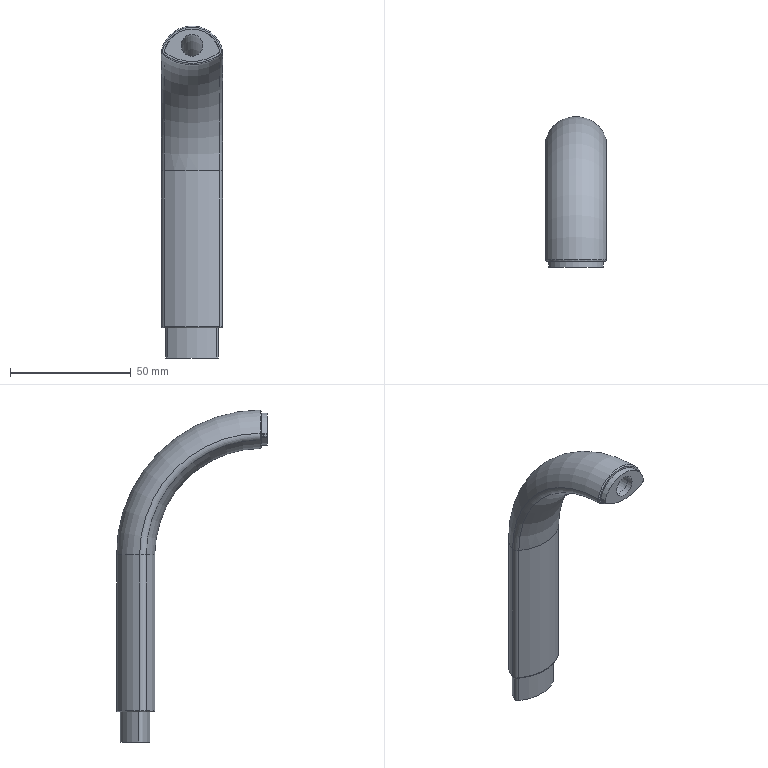Component | NX | ZHICHENGJIA | 1 solid | 49 faces | volume 37120 mm3 | cylinder 18 | plane 14 | torus 9 | spline 4 | cone 4 | commonest cylinder face diameters 3 x4 2.5 x2 5 x2 9 x2 11.25 x2 23.5 x1 23 x1 26 x1